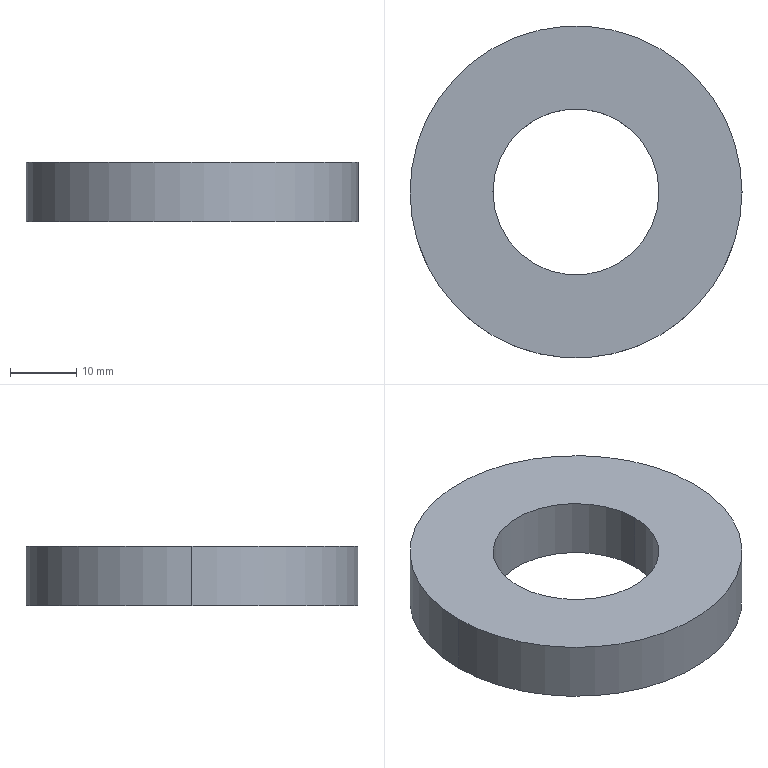Component | SolidWorks | Pulley-1 | 1 solid | 6 faces | box 50 x 50 x 9.02 mm | volume 13281 mm3 | cylinder 4 | plane 2 | commonest cylinder face diameters 25 x2 50 x2
build123d program:
from build123d import *

# Parameters (mm, degrees)
SKETCH1_R           = 25
SKETCH1_R_2         = 12.5
BOSS_EXTRUDE1_DEPTH = 17
MOVE_FACE1_BY       = 7.982


with BuildPart() as part:
    # Sketch1 → Boss-Extrude1 (new body)
    with BuildSketch(Plane.XY):
        Circle(SKETCH1_R)
        Circle(SKETCH1_R_2, mode=Mode.SUBTRACT)
    extrude(amount=-BOSS_EXTRUDE1_DEPTH)

    # Move Face1: a face moved inward by 7.981
    extrude(part.faces().sort_by_distance((0, -20, 0))[0], amount=MOVE_FACE1_BY, dir=(0, 0, -1), mode=Mode.SUBTRACT)


solid = part.part

# Placed as in the assembly
solid = solid.moved(Location((0, 0, -187.018), (0, 0, 0)))
STEP:
#1=CARTESIAN_POINT('',(0.4921,0.,-7.677));
#2=VERTEX_POINT('',#1);
#3=CARTESIAN_POINT('',(-0.4921,0.,-7.677));
#4=VERTEX_POINT('',#3);
#5=CARTESIAN_POINT('',(0.,0.,-7.677));
#6=DIRECTION('',(0.,0.,-1.));
#7=DIRECTION('',(-1.,0.,0.));
#8=AXIS2_PLACEMENT_3D('',#5,#6,#7);
#9=CIRCLE('',#8,0.4921);
#10=EDGE_CURVE('',#2,#4,#9,.T.);
#11=ORIENTED_EDGE('',*,*,#10,.F.);
#12=CARTESIAN_POINT('',(0.4921,0.,-8.032));
#13=VERTEX_POINT('',#12);
#14=CARTESIAN_POINT('',(0.4921,0.,-7.677));
#15=DIRECTION('',(0.,0.,-1.));
#16=VECTOR('',#15,39.37);
#17=LINE('',#14,#16);
#18=EDGE_CURVE('',#2,#13,#17,.T.);
#19=ORIENTED_EDGE('',*,*,#18,.T.);
#20=CARTESIAN_POINT('',(-0.4921,0.,-8.032));
#21=VERTEX_POINT('',#20);
#22=CARTESIAN_POINT('',(0.,0.,-8.032));
#23=DIRECTION('',(0.,0.,-1.));
#24=DIRECTION('',(-1.,0.,0.));
#25=AXIS2_PLACEMENT_3D('',#22,#23,#24);
#26=CIRCLE('',#25,0.4921);
#27=EDGE_CURVE('',#13,#21,#26,.T.);
#28=ORIENTED_EDGE('',*,*,#27,.T.);
#29=CARTESIAN_POINT('',(-0.4921,0.,-7.677));
#30=DIRECTION('',(0.,0.,-1.));
#31=VECTOR('',#30,39.37);
#32=LINE('',#29,#31);
#33=EDGE_CURVE('',#4,#21,#32,.T.);
#34=ORIENTED_EDGE('',*,*,#33,.F.);
#35=EDGE_LOOP('',(#11,#19,#28,#34));
#36=FACE_OUTER_BOUND('',#35,.T.);
#37=CARTESIAN_POINT('',(0.,0.,-7.677));
#38=DIRECTION('',(0.,0.,-1.));
#39=DIRECTION('',(-1.,0.,0.));
#40=AXIS2_PLACEMENT_3D('',#37,#38,#39);
#41=CYLINDRICAL_SURFACE('',#40,0.4921);
#42=ADVANCED_FACE('',(#36),#41,.F.);
#43=CARTESIAN_POINT('',(-0.9843,0.,-7.677));
#44=VERTEX_POINT('',#43);
#45=CARTESIAN_POINT('',(0.9843,0.,-7.677));
#46=VERTEX_POINT('',#45);
#47=CARTESIAN_POINT('',(0.,0.,-7.677));
#48=DIRECTION('',(0.,0.,-1.));
#49=DIRECTION('',(-1.,0.,0.));
#50=AXIS2_PLACEMENT_3D('',#47,#48,#49);
#51=CIRCLE('',#50,0.9843);
#52=EDGE_CURVE('',#44,#46,#51,.T.);
#53=ORIENTED_EDGE('',*,*,#52,.T.);
#54=CARTESIAN_POINT('',(0.9843,0.,-8.032));
#55=VERTEX_POINT('',#54);
#56=CARTESIAN_POINT('',(0.9843,0.,-7.677));
#57=DIRECTION('',(0.,0.,-1.));
#58=VECTOR('',#57,39.37);
#59=LINE('',#56,#58);
#60=EDGE_CURVE('',#46,#55,#59,.T.);
#61=ORIENTED_EDGE('',*,*,#60,.T.);
#62=CARTESIAN_POINT('',(-0.9843,0.,-8.032));
#63=VERTEX_POINT('',#62);
#64=CARTESIAN_POINT('',(0.,0.,-8.032));
#65=DIRECTION('',(0.,0.,-1.));
#66=DIRECTION('',(-1.,0.,0.));
#67=AXIS2_PLACEMENT_3D('',#64,#65,#66);
#68=CIRCLE('',#67,0.9843);
#69=EDGE_CURVE('',#63,#55,#68,.T.);
#70=ORIENTED_EDGE('',*,*,#69,.F.);
#71=CARTESIAN_POINT('',(-0.9843,0.,-7.677));
#72=DIRECTION('',(0.,0.,-1.));
#73=VECTOR('',#72,39.37);
#74=LINE('',#71,#73);
#75=EDGE_CURVE('',#44,#63,#74,.T.);
#76=ORIENTED_EDGE('',*,*,#75,.F.);
#77=EDGE_LOOP('',(#53,#61,#70,#76));
#78=FACE_OUTER_BOUND('',#77,.T.);
#79=CARTESIAN_POINT('',(0.,0.,-7.677));
#80=DIRECTION('',(0.,0.,-1.));
#81=DIRECTION('',(-1.,0.,0.));
#82=AXIS2_PLACEMENT_3D('',#79,#80,#81);
#83=CYLINDRICAL_SURFACE('',#82,0.9843);
#84=ADVANCED_FACE('',(#78),#83,.T.);
#85=ORIENTED_EDGE('',*,*,#60,.F.);
#86=CARTESIAN_POINT('',(0.,0.,-7.677));
#87=DIRECTION('',(0.,0.,-1.));
#88=DIRECTION('',(-1.,0.,0.));
#89=AXIS2_PLACEMENT_3D('',#86,#87,#88);
#90=CIRCLE('',#89,0.9843);
#91=EDGE_CURVE('',#46,#44,#90,.T.);
#92=ORIENTED_EDGE('',*,*,#91,.T.);
#93=ORIENTED_EDGE('',*,*,#75,.T.);
#94=CARTESIAN_POINT('',(0.,0.,-8.032));
#95=DIRECTION('',(0.,0.,-1.));
#96=DIRECTION('',(-1.,0.,0.));
#97=AXIS2_PLACEMENT_3D('',#94,#95,#96);
#98=CIRCLE('',#97,0.9843);
#99=EDGE_CURVE('',#55,#63,#98,.T.);
#100=ORIENTED_EDGE('',*,*,#99,.F.);
#101=EDGE_LOOP('',(#85,#92,#93,#100));
#102=FACE_OUTER_BOUND('',#101,.T.);
#103=CARTESIAN_POINT('',(0.,0.,-7.677));
#104=DIRECTION('',(0.,0.,-1.));
#105=DIRECTION('',(-1.,0.,0.));
#106=AXIS2_PLACEMENT_3D('',#103,#104,#105);
#107=CYLINDRICAL_SURFACE('',#106,0.9843);
#108=ADVANCED_FACE('',(#102),#107,.T.);
#109=CARTESIAN_POINT('',(0.,0.,-7.677));
#110=DIRECTION('',(0.,0.,-1.));
#111=DIRECTION('',(-1.,0.,0.));
#112=AXIS2_PLACEMENT_3D('',#109,#110,#111);
#113=CIRCLE('',#112,0.4921);
#114=EDGE_CURVE('',#4,#2,#113,.T.);
#115=ORIENTED_EDGE('',*,*,#114,.T.);
#116=ORIENTED_EDGE('',*,*,#10,.T.);
#117=EDGE_LOOP('',(#115,#116));
#118=FACE_BOUND('',#117,.T.);
#119=ORIENTED_EDGE('',*,*,#52,.F.);
#120=ORIENTED_EDGE('',*,*,#91,.F.);
#121=EDGE_LOOP('',(#119,#120));
#122=FACE_OUTER_BOUND('',#121,.T.);
#123=CARTESIAN_POINT('',(0.,0.,-7.677));
#124=DIRECTION('',(0.,0.,-1.));
#125=DIRECTION('',(-1.,0.,0.));
#126=AXIS2_PLACEMENT_3D('',#123,#124,#125);
#127=PLANE('',#126);
#128=ADVANCED_FACE('',(#118,#122),#127,.F.);
#129=CARTESIAN_POINT('',(0.,0.,-8.032));
#130=DIRECTION('',(0.,0.,-1.));
#131=DIRECTION('',(-1.,0.,0.));
#132=AXIS2_PLACEMENT_3D('',#129,#130,#131);
#133=CIRCLE('',#132,0.4921);
#134=EDGE_CURVE('',#21,#13,#133,.T.);
#135=ORIENTED_EDGE('',*,*,#134,.F.);
#136=ORIENTED_EDGE('',*,*,#27,.F.);
#137=EDGE_LOOP('',(#135,#136));
#138=FACE_BOUND('',#137,.T.);
#139=ORIENTED_EDGE('',*,*,#69,.T.);
#140=ORIENTED_EDGE('',*,*,#99,.T.);
#141=EDGE_LOOP('',(#139,#140));
#142=FACE_OUTER_BOUND('',#141,.T.);
#143=CARTESIAN_POINT('',(0.,0.,-8.032));
#144=DIRECTION('',(0.,0.,-1.));
#145=DIRECTION('',(-1.,0.,0.));
#146=AXIS2_PLACEMENT_3D('',#143,#144,#145);
#147=PLANE('',#146);
#148=ADVANCED_FACE('',(#138,#142),#147,.T.);
#149=ORIENTED_EDGE('',*,*,#18,.F.);
#150=ORIENTED_EDGE('',*,*,#114,.F.);
#151=ORIENTED_EDGE('',*,*,#33,.T.);
#152=ORIENTED_EDGE('',*,*,#134,.T.);
#153=EDGE_LOOP('',(#149,#150,#151,#152));
#154=FACE_OUTER_BOUND('',#153,.T.);
#155=CARTESIAN_POINT('',(0.,0.,-7.677));
#156=DIRECTION('',(0.,0.,-1.));
#157=DIRECTION('',(-1.,0.,0.));
#158=AXIS2_PLACEMENT_3D('',#155,#156,#157);
#159=CYLINDRICAL_SURFACE('',#158,0.4921);
#160=ADVANCED_FACE('',(#154),#159,.F.);
#161=CLOSED_SHELL('',(#42,#84,#108,#128,#148,#160));
#162=MANIFOLD_SOLID_BREP('',#161);
#163=CARTESIAN_POINT('',(0.,0.,0.));
#164=DIRECTION('',(0.,0.,1.));
#165=DIRECTION('',(1.,0.,0.));
#166=AXIS2_PLACEMENT_3D('',#163,#164,#165);
#167=(LENGTH_UNIT()NAMED_UNIT(*)SI_UNIT($,.METRE.));
#168=LENGTH_MEASURE_WITH_UNIT(LENGTH_MEASURE(0.0254),#167);
#169=DIMENSIONAL_EXPONENTS(1.,0.,0.,0.,0.,0.,0.);
#170=(CONVERSION_BASED_UNIT('',#168)LENGTH_UNIT()NAMED_UNIT(#169));
#171=UNCERTAINTY_MEASURE_WITH_UNIT(LENGTH_MEASURE(0.00001),#170,'','');
#172=(NAMED_UNIT(*)PLANE_ANGLE_UNIT()SI_UNIT($,.RADIAN.));
#173=(NAMED_UNIT(*)SI_UNIT($,.STERADIAN.)SOLID_ANGLE_UNIT());
#174=(GEOMETRIC_REPRESENTATION_CONTEXT(3)GLOBAL_UNCERTAINTY_ASSIGNED_CONTEXT((#171))GLOBAL_UNIT_ASSIGNED_CONTEXT((#170,#172,#173))REPRESENTATION_CONTEXT('',''));
#175=ADVANCED_BREP_SHAPE_REPRESENTATION('',(#162,#166),#174);
#176=COLOUR_RGB('',0.7922,0.8196,0.9333);
#177=FILL_AREA_STYLE_COLOUR('',#176);
#178=FILL_AREA_STYLE('',(#177));
#179=SURFACE_STYLE_FILL_AREA(#178);
#180=SURFACE_SIDE_STYLE('',(#179));
#181=SURFACE_STYLE_USAGE(.BOTH.,#180);
#182=PRESENTATION_STYLE_ASSIGNMENT((#181));
#183=STYLED_ITEM('',(#182),#162);
#184=(LENGTH_UNIT()NAMED_UNIT(*)SI_UNIT($,.METRE.));
#185=LENGTH_MEASURE_WITH_UNIT(LENGTH_MEASURE(0.0254),#184);
#186=DIMENSIONAL_EXPONENTS(1.,0.,0.,0.,0.,0.,0.);
#187=(CONVERSION_BASED_UNIT('',#185)LENGTH_UNIT()NAMED_UNIT(#186));
#188=UNCERTAINTY_MEASURE_WITH_UNIT(LENGTH_MEASURE(0.00001),#187,'','');
#189=(NAMED_UNIT(*)PLANE_ANGLE_UNIT()SI_UNIT($,.RADIAN.));
#190=(NAMED_UNIT(*)SI_UNIT($,.STERADIAN.)SOLID_ANGLE_UNIT());
#191=(GEOMETRIC_REPRESENTATION_CONTEXT(3)GLOBAL_UNCERTAINTY_ASSIGNED_CONTEXT((#188))GLOBAL_UNIT_ASSIGNED_CONTEXT((#187,#189,#190))REPRESENTATION_CONTEXT('',''));
#192=MECHANICAL_DESIGN_GEOMETRIC_PRESENTATION_REPRESENTATION('',(#183),#191);
#193=PRESENTATION_LAYER_ASSIGNMENT('','',(#183));